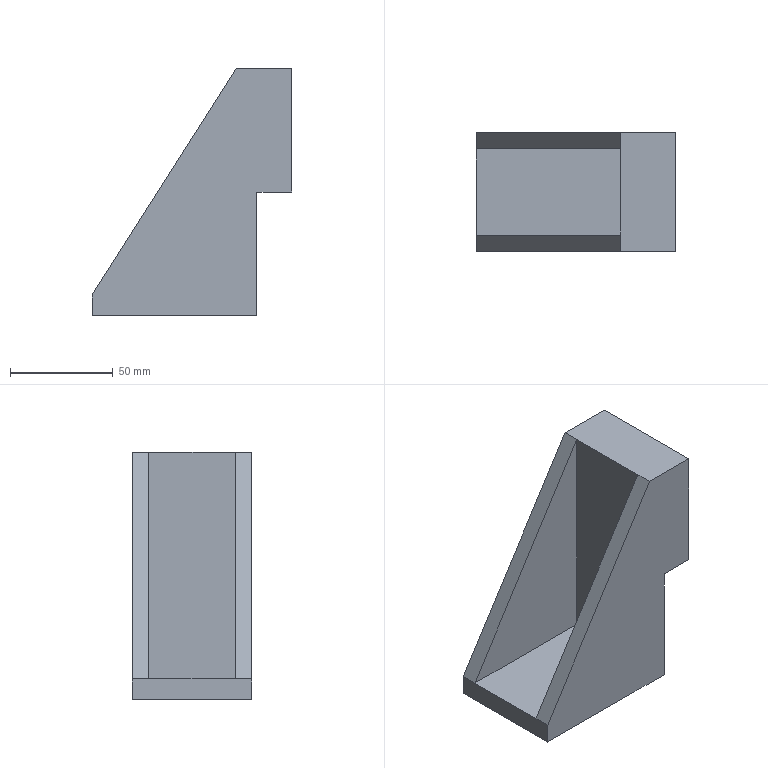Component | SolidWorks | 2023-12-12-29-1 | 1 solid | 14 faces | box 97 x 58 x 120 mm | volume 230960 mm3 | plane 14 | material AL6061
build123d program:
from build123d import *

# Parameters (mm, degrees)
BOSS_EXTRUDE1_DEPTH = 58
SKETCH2_W           = 42
SKETCH2_H           = 165.909
CUT_EXTRUDE1_DEPTH  = 70
SKETCH3_W           = 58
SKETCH3_H           = 60
BOSS_EXTRUDE2_DEPTH = 17


with BuildPart() as part:
    # Sketch1 → Boss-Extrude1 (new body)
    with BuildSketch(Plane.XY):
        Polygon((10, 120), (80, 10), (80, 0), (0, 0), (0, 120), align=None)
    extrude(amount=BOSS_EXTRUDE1_DEPTH)

    # Sketch2 → Cut-Extrude1 (cut)
    with BuildSketch(Plane(origin=(80, 0, 0), x_dir=(0, 0, -1), z_dir=(1, 0, 0))):
        with Locations((-29, 92.955)):
            Rectangle(SKETCH2_W, SKETCH2_H)
    extrude(amount=-CUT_EXTRUDE1_DEPTH, mode=Mode.SUBTRACT)

    # Sketch3 → Boss-Extrude2 (add)
    with BuildSketch(Plane.ZY):
        with Locations((29, 90)):
            Rectangle(SKETCH3_W, SKETCH3_H)
    extrude(amount=BOSS_EXTRUDE2_DEPTH)


solid = part.part

# Placed as in the assembly
solid = solid.moved(Location((-98.778, -31.867, 84), (-90, 0, 180)))
STEP:
#1=COLOUR_RGB('',0.7922,0.8196,0.9333);
#2=FILL_AREA_STYLE_COLOUR('',#1);
#3=FILL_AREA_STYLE('',(#2));
#4=SURFACE_STYLE_FILL_AREA(#3);
#5=SURFACE_SIDE_STYLE('',(#4));
#6=SURFACE_STYLE_USAGE(.BOTH.,#5);
#7=PRESENTATION_STYLE_ASSIGNMENT((#6));
#8=CARTESIAN_POINT('',(-3.889,-1.255,5.669));
#9=VERTEX_POINT('',#8);
#10=CARTESIAN_POINT('',(-3.889,1.029,5.669));
#11=VERTEX_POINT('',#10);
#12=CARTESIAN_POINT('',(-3.889,-1.255,5.669));
#13=DIRECTION('',(-0.,1.,-0.));
#14=VECTOR('',#13,39.37);
#15=LINE('',#12,#14);
#16=EDGE_CURVE('',#9,#11,#15,.T.);
#17=ORIENTED_EDGE('',*,*,#16,.F.);
#18=CARTESIAN_POINT('',(-3.889,-1.255,3.307));
#19=VERTEX_POINT('',#18);
#20=CARTESIAN_POINT('',(-3.889,-1.255,3.307));
#21=DIRECTION('',(0.,-0.,-1.));
#22=VECTOR('',#21,39.37);
#23=LINE('',#20,#22);
#24=EDGE_CURVE('',#9,#19,#23,.T.);
#25=ORIENTED_EDGE('',*,*,#24,.T.);
#26=CARTESIAN_POINT('',(-3.889,1.029,3.307));
#27=VERTEX_POINT('',#26);
#28=CARTESIAN_POINT('',(-3.889,1.029,3.307));
#29=DIRECTION('',(0.,-1.,0.));
#30=VECTOR('',#29,39.37);
#31=LINE('',#28,#30);
#32=EDGE_CURVE('',#27,#19,#31,.T.);
#33=ORIENTED_EDGE('',*,*,#32,.F.);
#34=CARTESIAN_POINT('',(-3.889,1.029,3.307));
#35=DIRECTION('',(0.,-0.,-1.));
#36=VECTOR('',#35,39.37);
#37=LINE('',#34,#36);
#38=EDGE_CURVE('',#11,#27,#37,.T.);
#39=ORIENTED_EDGE('',*,*,#38,.F.);
#40=EDGE_LOOP('',(#17,#25,#33,#39));
#41=FACE_OUTER_BOUND('',#40,.T.);
#42=CARTESIAN_POINT('',(-3.889,1.029,3.307));
#43=DIRECTION('',(-1.,-0.,-0.));
#44=DIRECTION('',(0.,-1.,0.));
#45=AXIS2_PLACEMENT_3D('',#42,#43,#44);
#46=PLANE('',#45);
#47=ADVANCED_FACE('',(#41),#46,.F.);
#48=CARTESIAN_POINT('',(-4.283,-0.9396,8.031));
#49=VERTEX_POINT('',#48);
#50=CARTESIAN_POINT('',(-4.283,-1.255,8.031));
#51=VERTEX_POINT('',#50);
#52=CARTESIAN_POINT('',(-4.283,1.029,8.031));
#53=DIRECTION('',(0.,-1.,0.));
#54=VECTOR('',#53,39.37);
#55=LINE('',#52,#54);
#56=EDGE_CURVE('',#49,#51,#55,.T.);
#57=ORIENTED_EDGE('',*,*,#56,.F.);
#58=CARTESIAN_POINT('',(-7.039,-0.9396,3.701));
#59=VERTEX_POINT('',#58);
#60=CARTESIAN_POINT('',(-4.283,-0.9396,8.031));
#61=DIRECTION('',(-0.5369,-0.,-0.8437));
#62=VECTOR('',#61,39.37);
#63=LINE('',#60,#62);
#64=EDGE_CURVE('',#49,#59,#63,.T.);
#65=ORIENTED_EDGE('',*,*,#64,.T.);
#66=CARTESIAN_POINT('',(-7.039,-1.255,3.701));
#67=VERTEX_POINT('',#66);
#68=CARTESIAN_POINT('',(-7.039,1.029,3.701));
#69=DIRECTION('',(0.,-1.,0.));
#70=VECTOR('',#69,39.37);
#71=LINE('',#68,#70);
#72=EDGE_CURVE('',#59,#67,#71,.T.);
#73=ORIENTED_EDGE('',*,*,#72,.T.);
#74=CARTESIAN_POINT('',(-4.283,-1.255,8.031));
#75=DIRECTION('',(0.5369,0.,0.8437));
#76=VECTOR('',#75,39.37);
#77=LINE('',#74,#76);
#78=EDGE_CURVE('',#67,#51,#77,.T.);
#79=ORIENTED_EDGE('',*,*,#78,.T.);
#80=EDGE_LOOP('',(#57,#65,#73,#79));
#81=FACE_OUTER_BOUND('',#80,.T.);
#82=CARTESIAN_POINT('',(-4.283,1.029,8.031));
#83=DIRECTION('',(0.8437,0.,-0.5369));
#84=DIRECTION('',(-0.5369,-0.,-0.8437));
#85=AXIS2_PLACEMENT_3D('',#82,#83,#84);
#86=PLANE('',#85);
#87=ADVANCED_FACE('',(#81),#86,.F.);
#88=CARTESIAN_POINT('',(-7.039,-1.255,3.307));
#89=VERTEX_POINT('',#88);
#90=CARTESIAN_POINT('',(-3.889,-1.255,3.307));
#91=DIRECTION('',(-1.,-0.,-0.));
#92=VECTOR('',#91,39.37);
#93=LINE('',#90,#92);
#94=EDGE_CURVE('',#19,#89,#93,.T.);
#95=ORIENTED_EDGE('',*,*,#94,.T.);
#96=CARTESIAN_POINT('',(-7.039,1.029,3.307));
#97=VERTEX_POINT('',#96);
#98=CARTESIAN_POINT('',(-7.039,1.029,3.307));
#99=DIRECTION('',(0.,-1.,0.));
#100=VECTOR('',#99,39.37);
#101=LINE('',#98,#100);
#102=EDGE_CURVE('',#97,#89,#101,.T.);
#103=ORIENTED_EDGE('',*,*,#102,.F.);
#104=CARTESIAN_POINT('',(-3.889,1.029,3.307));
#105=DIRECTION('',(-1.,-0.,-0.));
#106=VECTOR('',#105,39.37);
#107=LINE('',#104,#106);
#108=EDGE_CURVE('',#27,#97,#107,.T.);
#109=ORIENTED_EDGE('',*,*,#108,.F.);
#110=ORIENTED_EDGE('',*,*,#32,.T.);
#111=EDGE_LOOP('',(#95,#103,#109,#110));
#112=FACE_OUTER_BOUND('',#111,.T.);
#113=CARTESIAN_POINT('',(-3.889,1.029,3.307));
#114=DIRECTION('',(-0.,0.,1.));
#115=DIRECTION('',(-0.,1.,-0.));
#116=AXIS2_PLACEMENT_3D('',#113,#114,#115);
#117=PLANE('',#116);
#118=ADVANCED_FACE('',(#112),#117,.F.);
#119=CARTESIAN_POINT('',(-7.039,-1.255,3.307));
#120=DIRECTION('',(-0.,0.,1.));
#121=VECTOR('',#120,39.37);
#122=LINE('',#119,#121);
#123=EDGE_CURVE('',#89,#67,#122,.T.);
#124=ORIENTED_EDGE('',*,*,#123,.T.);
#125=ORIENTED_EDGE('',*,*,#72,.F.);
#126=CARTESIAN_POINT('',(-7.039,0.7139,3.701));
#127=VERTEX_POINT('',#126);
#128=CARTESIAN_POINT('',(-7.039,0.7139,3.701));
#129=DIRECTION('',(0.,-1.,0.));
#130=VECTOR('',#129,39.37);
#131=LINE('',#128,#130);
#132=EDGE_CURVE('',#127,#59,#131,.T.);
#133=ORIENTED_EDGE('',*,*,#132,.F.);
#134=CARTESIAN_POINT('',(-7.039,1.029,3.701));
#135=VERTEX_POINT('',#134);
#136=CARTESIAN_POINT('',(-7.039,1.029,3.701));
#137=DIRECTION('',(0.,-1.,0.));
#138=VECTOR('',#137,39.37);
#139=LINE('',#136,#138);
#140=EDGE_CURVE('',#135,#127,#139,.T.);
#141=ORIENTED_EDGE('',*,*,#140,.F.);
#142=CARTESIAN_POINT('',(-7.039,1.029,3.307));
#143=DIRECTION('',(-0.,0.,1.));
#144=VECTOR('',#143,39.37);
#145=LINE('',#142,#144);
#146=EDGE_CURVE('',#97,#135,#145,.T.);
#147=ORIENTED_EDGE('',*,*,#146,.F.);
#148=ORIENTED_EDGE('',*,*,#102,.T.);
#149=EDGE_LOOP('',(#124,#125,#133,#141,#147,#148));
#150=FACE_OUTER_BOUND('',#149,.T.);
#151=CARTESIAN_POINT('',(-7.039,1.029,3.307));
#152=DIRECTION('',(1.,0.,0.));
#153=DIRECTION('',(-0.,1.,-0.));
#154=AXIS2_PLACEMENT_3D('',#151,#152,#153);
#155=PLANE('',#154);
#156=ADVANCED_FACE('',(#150),#155,.F.);
#157=ORIENTED_EDGE('',*,*,#140,.T.);
#158=CARTESIAN_POINT('',(-4.283,0.7139,8.031));
#159=VERTEX_POINT('',#158);
#160=CARTESIAN_POINT('',(-4.283,0.7139,8.031));
#161=DIRECTION('',(0.5369,0.,0.8437));
#162=VECTOR('',#161,39.37);
#163=LINE('',#160,#162);
#164=EDGE_CURVE('',#127,#159,#163,.T.);
#165=ORIENTED_EDGE('',*,*,#164,.T.);
#166=CARTESIAN_POINT('',(-4.283,1.029,8.031));
#167=VERTEX_POINT('',#166);
#168=CARTESIAN_POINT('',(-4.283,1.029,8.031));
#169=DIRECTION('',(0.,-1.,0.));
#170=VECTOR('',#169,39.37);
#171=LINE('',#168,#170);
#172=EDGE_CURVE('',#167,#159,#171,.T.);
#173=ORIENTED_EDGE('',*,*,#172,.F.);
#174=CARTESIAN_POINT('',(-4.283,1.029,8.031));
#175=DIRECTION('',(0.5369,0.,0.8437));
#176=VECTOR('',#175,39.37);
#177=LINE('',#174,#176);
#178=EDGE_CURVE('',#135,#167,#177,.T.);
#179=ORIENTED_EDGE('',*,*,#178,.F.);
#180=EDGE_LOOP('',(#157,#165,#173,#179));
#181=FACE_OUTER_BOUND('',#180,.T.);
#182=CARTESIAN_POINT('',(-4.283,1.029,8.031));
#183=DIRECTION('',(0.8437,0.,-0.5369));
#184=DIRECTION('',(-0.5369,-0.,-0.8437));
#185=AXIS2_PLACEMENT_3D('',#182,#183,#184);
#186=PLANE('',#185);
#187=ADVANCED_FACE('',(#181),#186,.F.);
#188=CARTESIAN_POINT('',(-3.22,-1.255,8.031));
#189=VERTEX_POINT('',#188);
#190=CARTESIAN_POINT('',(-3.889,-1.255,8.031));
#191=DIRECTION('',(1.,0.,0.));
#192=VECTOR('',#191,39.37);
#193=LINE('',#190,#192);
#194=EDGE_CURVE('',#51,#189,#193,.T.);
#195=ORIENTED_EDGE('',*,*,#194,.T.);
#196=CARTESIAN_POINT('',(-3.22,1.029,8.031));
#197=VERTEX_POINT('',#196);
#198=CARTESIAN_POINT('',(-3.22,-1.255,8.031));
#199=DIRECTION('',(0.,-1.,0.));
#200=VECTOR('',#199,39.37);
#201=LINE('',#198,#200);
#202=EDGE_CURVE('',#197,#189,#201,.T.);
#203=ORIENTED_EDGE('',*,*,#202,.F.);
#204=CARTESIAN_POINT('',(-3.889,1.029,8.031));
#205=DIRECTION('',(1.,0.,0.));
#206=VECTOR('',#205,39.37);
#207=LINE('',#204,#206);
#208=EDGE_CURVE('',#167,#197,#207,.T.);
#209=ORIENTED_EDGE('',*,*,#208,.F.);
#210=ORIENTED_EDGE('',*,*,#172,.T.);
#211=CARTESIAN_POINT('',(-4.283,1.029,8.031));
#212=DIRECTION('',(0.,-1.,0.));
#213=VECTOR('',#212,39.37);
#214=LINE('',#211,#213);
#215=EDGE_CURVE('',#159,#49,#214,.T.);
#216=ORIENTED_EDGE('',*,*,#215,.T.);
#217=ORIENTED_EDGE('',*,*,#56,.T.);
#218=EDGE_LOOP('',(#195,#203,#209,#210,#216,#217));
#219=FACE_OUTER_BOUND('',#218,.T.);
#220=CARTESIAN_POINT('',(-3.889,1.029,8.031));
#221=DIRECTION('',(0.,-0.,-1.));
#222=DIRECTION('',(0.,-1.,0.));
#223=AXIS2_PLACEMENT_3D('',#220,#221,#222);
#224=PLANE('',#223);
#225=ADVANCED_FACE('',(#219),#224,.F.);
#226=ORIENTED_EDGE('',*,*,#208,.T.);
#227=CARTESIAN_POINT('',(-3.22,1.029,5.669));
#228=VERTEX_POINT('',#227);
#229=CARTESIAN_POINT('',(-3.22,1.029,8.031));
#230=DIRECTION('',(-0.,0.,1.));
#231=VECTOR('',#230,39.37);
#232=LINE('',#229,#231);
#233=EDGE_CURVE('',#228,#197,#232,.T.);
#234=ORIENTED_EDGE('',*,*,#233,.F.);
#235=CARTESIAN_POINT('',(-3.22,1.029,5.669));
#236=DIRECTION('',(-1.,-0.,-0.));
#237=VECTOR('',#236,39.37);
#238=LINE('',#235,#237);
#239=EDGE_CURVE('',#228,#11,#238,.T.);
#240=ORIENTED_EDGE('',*,*,#239,.T.);
#241=ORIENTED_EDGE('',*,*,#38,.T.);
#242=ORIENTED_EDGE('',*,*,#108,.T.);
#243=ORIENTED_EDGE('',*,*,#146,.T.);
#244=ORIENTED_EDGE('',*,*,#178,.T.);
#245=EDGE_LOOP('',(#226,#234,#240,#241,#242,#243,#244));
#246=FACE_OUTER_BOUND('',#245,.T.);
#247=CARTESIAN_POINT('',(-3.889,1.029,3.307));
#248=DIRECTION('',(0.,-1.,0.));
#249=DIRECTION('',(1.,0.,0.));
#250=AXIS2_PLACEMENT_3D('',#247,#248,#249);
#251=PLANE('',#250);
#252=ADVANCED_FACE('',(#246),#251,.F.);
#253=ORIENTED_EDGE('',*,*,#24,.F.);
#254=CARTESIAN_POINT('',(-3.22,-1.255,5.669));
#255=VERTEX_POINT('',#254);
#256=CARTESIAN_POINT('',(-3.22,-1.255,5.669));
#257=DIRECTION('',(-1.,-0.,-0.));
#258=VECTOR('',#257,39.37);
#259=LINE('',#256,#258);
#260=EDGE_CURVE('',#255,#9,#259,.T.);
#261=ORIENTED_EDGE('',*,*,#260,.F.);
#262=CARTESIAN_POINT('',(-3.22,-1.255,8.031));
#263=DIRECTION('',(0.,-0.,-1.));
#264=VECTOR('',#263,39.37);
#265=LINE('',#262,#264);
#266=EDGE_CURVE('',#189,#255,#265,.T.);
#267=ORIENTED_EDGE('',*,*,#266,.F.);
#268=ORIENTED_EDGE('',*,*,#194,.F.);
#269=ORIENTED_EDGE('',*,*,#78,.F.);
#270=ORIENTED_EDGE('',*,*,#123,.F.);
#271=ORIENTED_EDGE('',*,*,#94,.F.);
#272=EDGE_LOOP('',(#253,#261,#267,#268,#269,#270,#271));
#273=FACE_OUTER_BOUND('',#272,.T.);
#274=CARTESIAN_POINT('',(-3.889,-1.255,3.307));
#275=DIRECTION('',(0.,-1.,0.));
#276=DIRECTION('',(1.,0.,0.));
#277=AXIS2_PLACEMENT_3D('',#274,#275,#276);
#278=PLANE('',#277);
#279=ADVANCED_FACE('',(#273),#278,.T.);
#280=CARTESIAN_POINT('',(-4.283,-0.9396,3.701));
#281=VERTEX_POINT('',#280);
#282=CARTESIAN_POINT('',(-4.283,-0.9396,10.233));
#283=DIRECTION('',(-0.,0.,1.));
#284=VECTOR('',#283,39.37);
#285=LINE('',#282,#284);
#286=EDGE_CURVE('',#281,#49,#285,.T.);
#287=ORIENTED_EDGE('',*,*,#286,.F.);
#288=CARTESIAN_POINT('',(-4.283,-0.9396,3.701));
#289=DIRECTION('',(-1.,-0.,-0.));
#290=VECTOR('',#289,39.37);
#291=LINE('',#288,#290);
#292=EDGE_CURVE('',#281,#59,#291,.T.);
#293=ORIENTED_EDGE('',*,*,#292,.T.);
#294=ORIENTED_EDGE('',*,*,#64,.F.);
#295=EDGE_LOOP('',(#287,#293,#294));
#296=FACE_OUTER_BOUND('',#295,.T.);
#297=CARTESIAN_POINT('',(-4.283,-0.9396,10.233));
#298=DIRECTION('',(0.,-1.,0.));
#299=DIRECTION('',(1.,0.,0.));
#300=AXIS2_PLACEMENT_3D('',#297,#298,#299);
#301=PLANE('',#300);
#302=ADVANCED_FACE('',(#296),#301,.F.);
#303=CARTESIAN_POINT('',(-4.283,0.7139,3.701));
#304=VERTEX_POINT('',#303);
#305=CARTESIAN_POINT('',(-4.283,0.7139,3.701));
#306=DIRECTION('',(-1.,-0.,-0.));
#307=VECTOR('',#306,39.37);
#308=LINE('',#305,#307);
#309=EDGE_CURVE('',#304,#127,#308,.T.);
#310=ORIENTED_EDGE('',*,*,#309,.F.);
#311=CARTESIAN_POINT('',(-4.283,0.7139,10.233));
#312=DIRECTION('',(0.,-0.,-1.));
#313=VECTOR('',#312,39.37);
#314=LINE('',#311,#313);
#315=EDGE_CURVE('',#159,#304,#314,.T.);
#316=ORIENTED_EDGE('',*,*,#315,.F.);
#317=ORIENTED_EDGE('',*,*,#164,.F.);
#318=EDGE_LOOP('',(#310,#316,#317));
#319=FACE_OUTER_BOUND('',#318,.T.);
#320=CARTESIAN_POINT('',(-4.283,0.7139,10.233));
#321=DIRECTION('',(-0.,1.,-0.));
#322=DIRECTION('',(0.,-0.,-1.));
#323=AXIS2_PLACEMENT_3D('',#320,#321,#322);
#324=PLANE('',#323);
#325=ADVANCED_FACE('',(#319),#324,.F.);
#326=ORIENTED_EDGE('',*,*,#215,.F.);
#327=ORIENTED_EDGE('',*,*,#315,.T.);
#328=CARTESIAN_POINT('',(-4.283,0.7139,3.701));
#329=DIRECTION('',(0.,-1.,0.));
#330=VECTOR('',#329,39.37);
#331=LINE('',#328,#330);
#332=EDGE_CURVE('',#304,#281,#331,.T.);
#333=ORIENTED_EDGE('',*,*,#332,.T.);
#334=ORIENTED_EDGE('',*,*,#286,.T.);
#335=EDGE_LOOP('',(#326,#327,#333,#334));
#336=FACE_OUTER_BOUND('',#335,.T.);
#337=CARTESIAN_POINT('',(-4.283,-1.255,3.307));
#338=DIRECTION('',(-1.,-0.,-0.));
#339=DIRECTION('',(0.,-1.,0.));
#340=AXIS2_PLACEMENT_3D('',#337,#338,#339);
#341=PLANE('',#340);
#342=ADVANCED_FACE('',(#336),#341,.T.);
#343=ORIENTED_EDGE('',*,*,#132,.T.);
#344=ORIENTED_EDGE('',*,*,#292,.F.);
#345=ORIENTED_EDGE('',*,*,#332,.F.);
#346=ORIENTED_EDGE('',*,*,#309,.T.);
#347=EDGE_LOOP('',(#343,#344,#345,#346));
#348=FACE_OUTER_BOUND('',#347,.T.);
#349=CARTESIAN_POINT('',(-4.283,0.7139,3.701));
#350=DIRECTION('',(0.,-0.,-1.));
#351=DIRECTION('',(0.,-1.,0.));
#352=AXIS2_PLACEMENT_3D('',#349,#350,#351);
#353=PLANE('',#352);
#354=ADVANCED_FACE('',(#348),#353,.F.);
#355=ORIENTED_EDGE('',*,*,#16,.T.);
#356=ORIENTED_EDGE('',*,*,#239,.F.);
#357=CARTESIAN_POINT('',(-3.22,-1.255,5.669));
#358=DIRECTION('',(-0.,1.,-0.));
#359=VECTOR('',#358,39.37);
#360=LINE('',#357,#359);
#361=EDGE_CURVE('',#255,#228,#360,.T.);
#362=ORIENTED_EDGE('',*,*,#361,.F.);
#363=ORIENTED_EDGE('',*,*,#260,.T.);
#364=EDGE_LOOP('',(#355,#356,#362,#363));
#365=FACE_OUTER_BOUND('',#364,.T.);
#366=CARTESIAN_POINT('',(-3.22,-1.255,5.669));
#367=DIRECTION('',(-0.,0.,1.));
#368=DIRECTION('',(-0.,1.,-0.));
#369=AXIS2_PLACEMENT_3D('',#366,#367,#368);
#370=PLANE('',#369);
#371=ADVANCED_FACE('',(#365),#370,.F.);
#372=ORIENTED_EDGE('',*,*,#266,.T.);
#373=ORIENTED_EDGE('',*,*,#361,.T.);
#374=ORIENTED_EDGE('',*,*,#233,.T.);
#375=ORIENTED_EDGE('',*,*,#202,.T.);
#376=EDGE_LOOP('',(#372,#373,#374,#375));
#377=FACE_OUTER_BOUND('',#376,.T.);
#378=CARTESIAN_POINT('',(-3.22,-1.255,3.307));
#379=DIRECTION('',(1.,0.,0.));
#380=DIRECTION('',(-0.,1.,-0.));
#381=AXIS2_PLACEMENT_3D('',#378,#379,#380);
#382=PLANE('',#381);
#383=ADVANCED_FACE('',(#377),#382,.T.);
#384=CLOSED_SHELL('',(#47,#87,#118,#156,#187,#225,#252,#279,#302,#325,#342,#354,#371,#383));
#385=MANIFOLD_SOLID_BREP('',#384);
#386=STYLED_ITEM('',(#7),#385);
#387=(LENGTH_UNIT()NAMED_UNIT(*)SI_UNIT($,.METRE.));
#388=LENGTH_MEASURE_WITH_UNIT(LENGTH_MEASURE(0.0254),#387);
#389=DIMENSIONAL_EXPONENTS(1.,0.,0.,0.,0.,0.,0.);
#390=(CONVERSION_BASED_UNIT('',#388)LENGTH_UNIT()NAMED_UNIT(#389));
#391=UNCERTAINTY_MEASURE_WITH_UNIT(LENGTH_MEASURE(0.00001),#390,'','');
#392=(NAMED_UNIT(*)PLANE_ANGLE_UNIT()SI_UNIT($,.RADIAN.));
#393=(NAMED_UNIT(*)SI_UNIT($,.STERADIAN.)SOLID_ANGLE_UNIT());
#394=(GEOMETRIC_REPRESENTATION_CONTEXT(3)GLOBAL_UNCERTAINTY_ASSIGNED_CONTEXT((#391))GLOBAL_UNIT_ASSIGNED_CONTEXT((#390,#392,#393))REPRESENTATION_CONTEXT('',''));
#395=MECHANICAL_DESIGN_GEOMETRIC_PRESENTATION_REPRESENTATION('',(#386),#394);
#396=CARTESIAN_POINT('',(0.,0.,0.));
#397=DIRECTION('',(0.,0.,1.));
#398=DIRECTION('',(1.,0.,0.));
#399=AXIS2_PLACEMENT_3D('',#396,#397,#398);
#400=(LENGTH_UNIT()NAMED_UNIT(*)SI_UNIT($,.METRE.));
#401=LENGTH_MEASURE_WITH_UNIT(LENGTH_MEASURE(0.0254),#400);
#402=DIMENSIONAL_EXPONENTS(1.,0.,0.,0.,0.,0.,0.);
#403=(CONVERSION_BASED_UNIT('',#401)LENGTH_UNIT()NAMED_UNIT(#402));
#404=UNCERTAINTY_MEASURE_WITH_UNIT(LENGTH_MEASURE(0.00001),#403,'','');
#405=(NAMED_UNIT(*)PLANE_ANGLE_UNIT()SI_UNIT($,.RADIAN.));
#406=(NAMED_UNIT(*)SI_UNIT($,.STERADIAN.)SOLID_ANGLE_UNIT());
#407=(GEOMETRIC_REPRESENTATION_CONTEXT(3)GLOBAL_UNCERTAINTY_ASSIGNED_CONTEXT((#404))GLOBAL_UNIT_ASSIGNED_CONTEXT((#403,#405,#406))REPRESENTATION_CONTEXT('',''));
#408=ADVANCED_BREP_SHAPE_REPRESENTATION('',(#385,#399),#407);
#409=PRESENTATION_LAYER_ASSIGNMENT('','',(#386));